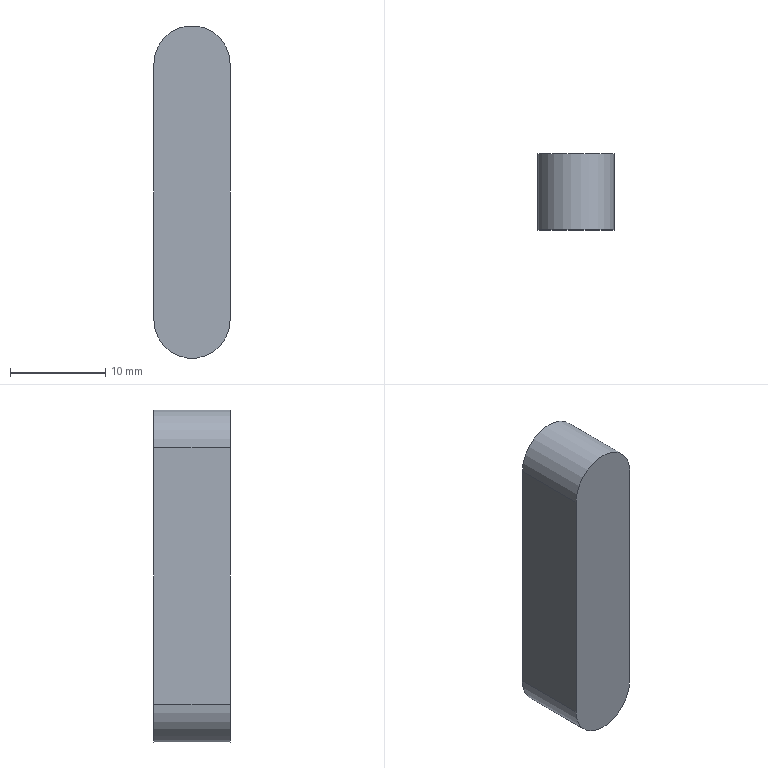Component | NX | FLAT_KEY_2 | 1 solid | 6 faces | box 8 x 8 x 35 mm | volume 2130 mm3 | plane 4 | cylinder 2 | commonest cylinder face diameters 8 x2
STEP:
#1=CARTESIAN_POINT('',(0.,0.,0.));
#2=DIRECTION('',(0.,0.,1.));
#3=DIRECTION('',(1.,0.,0.));
#4=AXIS2_PLACEMENT_3D('',#1,#2,#3);
#5=CARTESIAN_POINT('',(-515.175,316.681,-714.));
#6=VERTEX_POINT('',#5);
#7=CARTESIAN_POINT('',(-515.175,316.681,-687.));
#8=VERTEX_POINT('',#7);
#9=CARTESIAN_POINT('',(-515.175,316.681,-700.5));
#10=DIRECTION('',(0.,0.,1.));
#11=VECTOR('',#10,1.);
#12=LINE('',#9,#11);
#13=CARTESIAN_POINT('',(-511.175,316.681,-700.5));
#14=DIRECTION('',(0.,-1.,0.));
#15=DIRECTION('',(0.,0.,-1.));
#16=AXIS2_PLACEMENT_3D('',#13,#14,#15);
#17=PLANE('',#16);
#18=CARTESIAN_POINT('',(0.,-4.));
#19=DIRECTION('',(-1.,0.));
#20=VECTOR('',#19,1.);
#21=LINE('',#18,#20);
#22=(GEOMETRIC_REPRESENTATION_CONTEXT(2)PARAMETRIC_REPRESENTATION_CONTEXT()REPRESENTATION_CONTEXT('',''));
#23=DEFINITIONAL_REPRESENTATION('',(#21),#22);
#24=PCURVE('',#17,#23);
#25=CARTESIAN_POINT('',(-515.175,324.681,-700.5));
#26=DIRECTION('',(-1.,0.,0.));
#27=DIRECTION('',(0.,1.,0.));
#28=AXIS2_PLACEMENT_3D('',#25,#26,#27);
#29=PLANE('',#28);
#30=CARTESIAN_POINT('',(-8.,0.));
#31=DIRECTION('',(0.,-1.));
#32=VECTOR('',#31,1.);
#33=LINE('',#30,#32);
#34=(GEOMETRIC_REPRESENTATION_CONTEXT(2)PARAMETRIC_REPRESENTATION_CONTEXT()REPRESENTATION_CONTEXT('',''));
#35=DEFINITIONAL_REPRESENTATION('',(#33),#34);
#36=PCURVE('',#29,#35);
#37=SURFACE_CURVE('',#12,(#24,#36),.PCURVE_S1.);
#38=EDGE_CURVE('',#6,#8,#37,.T.);
#39=ORIENTED_EDGE('',*,*,#38,.F.);
#40=CARTESIAN_POINT('',(-507.175,316.681,-714.));
#41=VERTEX_POINT('',#40);
#42=CARTESIAN_POINT('',(-511.175,316.681,-714.));
#43=DIRECTION('',(0.,-1.,0.));
#44=DIRECTION('',(0.,0.,-1.));
#45=AXIS2_PLACEMENT_3D('',#42,#43,#44);
#46=CIRCLE('',#45,4.);
#47=CARTESIAN_POINT('',(13.5,0.));
#48=DIRECTION('',(1.,0.));
#49=AXIS2_PLACEMENT_2D('',#47,#48);
#50=CIRCLE('',#49,4.);
#51=(GEOMETRIC_REPRESENTATION_CONTEXT(2)PARAMETRIC_REPRESENTATION_CONTEXT()REPRESENTATION_CONTEXT('',''));
#52=DEFINITIONAL_REPRESENTATION('',(#50),#51);
#53=PCURVE('',#17,#52);
#54=CARTESIAN_POINT('',(-511.175,324.681,-714.));
#55=DIRECTION('',(0.,-1.,0.));
#56=DIRECTION('',(0.,0.,-1.));
#57=AXIS2_PLACEMENT_3D('',#54,#55,#56);
#58=CYLINDRICAL_SURFACE('',#57,4.);
#59=CARTESIAN_POINT('',(0.,8.));
#60=DIRECTION('',(1.,0.));
#61=VECTOR('',#60,1.);
#62=LINE('',#59,#61);
#63=(GEOMETRIC_REPRESENTATION_CONTEXT(2)PARAMETRIC_REPRESENTATION_CONTEXT()REPRESENTATION_CONTEXT('',''));
#64=DEFINITIONAL_REPRESENTATION('',(#62),#63);
#65=PCURVE('',#58,#64);
#66=SURFACE_CURVE('',#46,(#53,#65),.PCURVE_S1.);
#67=EDGE_CURVE('',#6,#41,#66,.T.);
#68=ORIENTED_EDGE('',*,*,#67,.T.);
#69=CARTESIAN_POINT('',(-507.175,316.681,-687.));
#70=VERTEX_POINT('',#69);
#71=CARTESIAN_POINT('',(-507.175,316.681,-700.5));
#72=DIRECTION('',(0.,0.,-1.));
#73=VECTOR('',#72,1.);
#74=LINE('',#71,#73);
#75=CARTESIAN_POINT('',(0.,4.));
#76=DIRECTION('',(1.,0.));
#77=VECTOR('',#76,1.);
#78=LINE('',#75,#77);
#79=(GEOMETRIC_REPRESENTATION_CONTEXT(2)PARAMETRIC_REPRESENTATION_CONTEXT()REPRESENTATION_CONTEXT('',''));
#80=DEFINITIONAL_REPRESENTATION('',(#78),#79);
#81=PCURVE('',#17,#80);
#82=CARTESIAN_POINT('',(-507.175,324.681,-700.5));
#83=DIRECTION('',(1.,0.,0.));
#84=DIRECTION('',(0.,-1.,0.));
#85=AXIS2_PLACEMENT_3D('',#82,#83,#84);
#86=PLANE('',#85);
#87=CARTESIAN_POINT('',(8.,0.));
#88=DIRECTION('',(0.,1.));
#89=VECTOR('',#88,1.);
#90=LINE('',#87,#89);
#91=(GEOMETRIC_REPRESENTATION_CONTEXT(2)PARAMETRIC_REPRESENTATION_CONTEXT()REPRESENTATION_CONTEXT('',''));
#92=DEFINITIONAL_REPRESENTATION('',(#90),#91);
#93=PCURVE('',#86,#92);
#94=SURFACE_CURVE('',#74,(#81,#93),.PCURVE_S1.);
#95=EDGE_CURVE('',#70,#41,#94,.T.);
#96=ORIENTED_EDGE('',*,*,#95,.F.);
#97=CARTESIAN_POINT('',(-511.175,316.681,-687.));
#98=DIRECTION('',(0.,-1.,0.));
#99=DIRECTION('',(0.,0.,-1.));
#100=AXIS2_PLACEMENT_3D('',#97,#98,#99);
#101=CIRCLE('',#100,4.);
#102=CARTESIAN_POINT('',(-13.5,0.));
#103=DIRECTION('',(1.,0.));
#104=AXIS2_PLACEMENT_2D('',#102,#103);
#105=CIRCLE('',#104,4.);
#106=(GEOMETRIC_REPRESENTATION_CONTEXT(2)PARAMETRIC_REPRESENTATION_CONTEXT()REPRESENTATION_CONTEXT('',''));
#107=DEFINITIONAL_REPRESENTATION('',(#105),#106);
#108=PCURVE('',#17,#107);
#109=CARTESIAN_POINT('',(-511.175,324.681,-687.));
#110=DIRECTION('',(0.,-1.,0.));
#111=DIRECTION('',(0.,0.,-1.));
#112=AXIS2_PLACEMENT_3D('',#109,#110,#111);
#113=CYLINDRICAL_SURFACE('',#112,4.);
#114=CARTESIAN_POINT('',(0.,8.));
#115=DIRECTION('',(1.,0.));
#116=VECTOR('',#115,1.);
#117=LINE('',#114,#116);
#118=(GEOMETRIC_REPRESENTATION_CONTEXT(2)PARAMETRIC_REPRESENTATION_CONTEXT()REPRESENTATION_CONTEXT('',''));
#119=DEFINITIONAL_REPRESENTATION('',(#117),#118);
#120=PCURVE('',#113,#119);
#121=SURFACE_CURVE('',#101,(#108,#120),.PCURVE_S1.);
#122=EDGE_CURVE('',#70,#8,#121,.T.);
#123=ORIENTED_EDGE('',*,*,#122,.T.);
#124=EDGE_LOOP('',(#39,#68,#96,#123));
#125=FACE_BOUND('',#124,.T.);
#126=ADVANCED_FACE('',(#125),#17,.T.);
#127=CARTESIAN_POINT('',(-515.175,324.681,-687.));
#128=VERTEX_POINT('',#127);
#129=CARTESIAN_POINT('',(-515.175,324.681,-714.));
#130=VERTEX_POINT('',#129);
#131=CARTESIAN_POINT('',(-515.175,324.681,-700.5));
#132=DIRECTION('',(0.,0.,-1.));
#133=VECTOR('',#132,1.);
#134=LINE('',#131,#133);
#135=CARTESIAN_POINT('',(0.,0.));
#136=DIRECTION('',(0.,1.));
#137=VECTOR('',#136,1.);
#138=LINE('',#135,#137);
#139=(GEOMETRIC_REPRESENTATION_CONTEXT(2)PARAMETRIC_REPRESENTATION_CONTEXT()REPRESENTATION_CONTEXT('',''));
#140=DEFINITIONAL_REPRESENTATION('',(#138),#139);
#141=PCURVE('',#29,#140);
#142=CARTESIAN_POINT('',(-511.175,324.681,-700.5));
#143=DIRECTION('',(0.,1.,0.));
#144=DIRECTION('',(0.,0.,1.));
#145=AXIS2_PLACEMENT_3D('',#142,#143,#144);
#146=PLANE('',#145);
#147=CARTESIAN_POINT('',(0.,-4.));
#148=DIRECTION('',(-1.,0.));
#149=VECTOR('',#148,1.);
#150=LINE('',#147,#149);
#151=(GEOMETRIC_REPRESENTATION_CONTEXT(2)PARAMETRIC_REPRESENTATION_CONTEXT()REPRESENTATION_CONTEXT('',''));
#152=DEFINITIONAL_REPRESENTATION('',(#150),#151);
#153=PCURVE('',#146,#152);
#154=SURFACE_CURVE('',#134,(#141,#153),.PCURVE_S1.);
#155=EDGE_CURVE('',#128,#130,#154,.T.);
#156=ORIENTED_EDGE('',*,*,#155,.T.);
#157=CARTESIAN_POINT('',(-515.175,324.681,-714.));
#158=DIRECTION('',(0.,-1.,0.));
#159=VECTOR('',#158,1.);
#160=LINE('',#157,#159);
#161=CARTESIAN_POINT('',(0.,13.5));
#162=DIRECTION('',(-1.,0.));
#163=VECTOR('',#162,1.);
#164=LINE('',#161,#163);
#165=(GEOMETRIC_REPRESENTATION_CONTEXT(2)PARAMETRIC_REPRESENTATION_CONTEXT()REPRESENTATION_CONTEXT('',''));
#166=DEFINITIONAL_REPRESENTATION('',(#164),#165);
#167=PCURVE('',#29,#166);
#168=CARTESIAN_POINT('',(4.712,0.));
#169=DIRECTION('',(0.,1.));
#170=VECTOR('',#169,1.);
#171=LINE('',#168,#170);
#172=(GEOMETRIC_REPRESENTATION_CONTEXT(2)PARAMETRIC_REPRESENTATION_CONTEXT()REPRESENTATION_CONTEXT('',''));
#173=DEFINITIONAL_REPRESENTATION('',(#171),#172);
#174=PCURVE('',#58,#173);
#175=SURFACE_CURVE('',#160,(#167,#174),.PCURVE_S1.);
#176=EDGE_CURVE('',#130,#6,#175,.T.);
#177=ORIENTED_EDGE('',*,*,#176,.T.);
#178=ORIENTED_EDGE('',*,*,#38,.T.);
#179=CARTESIAN_POINT('',(-515.175,324.681,-687.));
#180=DIRECTION('',(0.,1.,0.));
#181=VECTOR('',#180,1.);
#182=LINE('',#179,#181);
#183=CARTESIAN_POINT('',(0.,-13.5));
#184=DIRECTION('',(1.,0.));
#185=VECTOR('',#184,1.);
#186=LINE('',#183,#185);
#187=(GEOMETRIC_REPRESENTATION_CONTEXT(2)PARAMETRIC_REPRESENTATION_CONTEXT()REPRESENTATION_CONTEXT('',''));
#188=DEFINITIONAL_REPRESENTATION('',(#186),#187);
#189=PCURVE('',#29,#188);
#190=CARTESIAN_POINT('',(4.712,0.));
#191=DIRECTION('',(0.,-1.));
#192=VECTOR('',#191,1.);
#193=LINE('',#190,#192);
#194=(GEOMETRIC_REPRESENTATION_CONTEXT(2)PARAMETRIC_REPRESENTATION_CONTEXT()REPRESENTATION_CONTEXT('',''));
#195=DEFINITIONAL_REPRESENTATION('',(#193),#194);
#196=PCURVE('',#113,#195);
#197=SURFACE_CURVE('',#182,(#189,#196),.PCURVE_S1.);
#198=EDGE_CURVE('',#8,#128,#197,.T.);
#199=ORIENTED_EDGE('',*,*,#198,.T.);
#200=EDGE_LOOP('',(#156,#177,#178,#199));
#201=FACE_BOUND('',#200,.T.);
#202=ADVANCED_FACE('',(#201),#29,.T.);
#203=ORIENTED_EDGE('',*,*,#95,.T.);
#204=CARTESIAN_POINT('',(-507.175,324.681,-714.));
#205=VERTEX_POINT('',#204);
#206=CARTESIAN_POINT('',(-507.175,324.681,-714.));
#207=DIRECTION('',(0.,1.,0.));
#208=VECTOR('',#207,1.);
#209=LINE('',#206,#208);
#210=CARTESIAN_POINT('',(0.,13.5));
#211=DIRECTION('',(-1.,0.));
#212=VECTOR('',#211,1.);
#213=LINE('',#210,#212);
#214=(GEOMETRIC_REPRESENTATION_CONTEXT(2)PARAMETRIC_REPRESENTATION_CONTEXT()REPRESENTATION_CONTEXT('',''));
#215=DEFINITIONAL_REPRESENTATION('',(#213),#214);
#216=PCURVE('',#86,#215);
#217=CARTESIAN_POINT('',(7.854,0.));
#218=DIRECTION('',(0.,-1.));
#219=VECTOR('',#218,1.);
#220=LINE('',#217,#219);
#221=(GEOMETRIC_REPRESENTATION_CONTEXT(2)PARAMETRIC_REPRESENTATION_CONTEXT()REPRESENTATION_CONTEXT('',''));
#222=DEFINITIONAL_REPRESENTATION('',(#220),#221);
#223=PCURVE('',#58,#222);
#224=SURFACE_CURVE('',#209,(#216,#223),.PCURVE_S1.);
#225=EDGE_CURVE('',#41,#205,#224,.T.);
#226=ORIENTED_EDGE('',*,*,#225,.T.);
#227=CARTESIAN_POINT('',(-507.175,324.681,-687.));
#228=VERTEX_POINT('',#227);
#229=CARTESIAN_POINT('',(-507.175,324.681,-700.5));
#230=DIRECTION('',(0.,0.,1.));
#231=VECTOR('',#230,1.);
#232=LINE('',#229,#231);
#233=CARTESIAN_POINT('',(0.,0.));
#234=DIRECTION('',(0.,-1.));
#235=VECTOR('',#234,1.);
#236=LINE('',#233,#235);
#237=(GEOMETRIC_REPRESENTATION_CONTEXT(2)PARAMETRIC_REPRESENTATION_CONTEXT()REPRESENTATION_CONTEXT('',''));
#238=DEFINITIONAL_REPRESENTATION('',(#236),#237);
#239=PCURVE('',#86,#238);
#240=CARTESIAN_POINT('',(0.,4.));
#241=DIRECTION('',(1.,0.));
#242=VECTOR('',#241,1.);
#243=LINE('',#240,#242);
#244=(GEOMETRIC_REPRESENTATION_CONTEXT(2)PARAMETRIC_REPRESENTATION_CONTEXT()REPRESENTATION_CONTEXT('',''));
#245=DEFINITIONAL_REPRESENTATION('',(#243),#244);
#246=PCURVE('',#146,#245);
#247=SURFACE_CURVE('',#232,(#239,#246),.PCURVE_S1.);
#248=EDGE_CURVE('',#205,#228,#247,.T.);
#249=ORIENTED_EDGE('',*,*,#248,.T.);
#250=CARTESIAN_POINT('',(-507.175,324.681,-687.));
#251=DIRECTION('',(0.,-1.,0.));
#252=VECTOR('',#251,1.);
#253=LINE('',#250,#252);
#254=CARTESIAN_POINT('',(0.,-13.5));
#255=DIRECTION('',(1.,0.));
#256=VECTOR('',#255,1.);
#257=LINE('',#254,#256);
#258=(GEOMETRIC_REPRESENTATION_CONTEXT(2)PARAMETRIC_REPRESENTATION_CONTEXT()REPRESENTATION_CONTEXT('',''));
#259=DEFINITIONAL_REPRESENTATION('',(#257),#258);
#260=PCURVE('',#86,#259);
#261=CARTESIAN_POINT('',(1.571,0.));
#262=DIRECTION('',(0.,1.));
#263=VECTOR('',#262,1.);
#264=LINE('',#261,#263);
#265=(GEOMETRIC_REPRESENTATION_CONTEXT(2)PARAMETRIC_REPRESENTATION_CONTEXT()REPRESENTATION_CONTEXT('',''));
#266=DEFINITIONAL_REPRESENTATION('',(#264),#265);
#267=PCURVE('',#113,#266);
#268=SURFACE_CURVE('',#253,(#260,#267),.PCURVE_S1.);
#269=EDGE_CURVE('',#228,#70,#268,.T.);
#270=ORIENTED_EDGE('',*,*,#269,.T.);
#271=EDGE_LOOP('',(#203,#226,#249,#270));
#272=FACE_BOUND('',#271,.T.);
#273=ADVANCED_FACE('',(#272),#86,.T.);
#274=CARTESIAN_POINT('',(-511.175,324.681,-714.));
#275=DIRECTION('',(0.,1.,0.));
#276=DIRECTION('',(0.,0.,1.));
#277=AXIS2_PLACEMENT_3D('',#274,#275,#276);
#278=CIRCLE('',#277,4.);
#279=CARTESIAN_POINT('',(-13.5,0.));
#280=DIRECTION('',(1.,0.));
#281=AXIS2_PLACEMENT_2D('',#279,#280);
#282=CIRCLE('',#281,4.);
#283=(GEOMETRIC_REPRESENTATION_CONTEXT(2)PARAMETRIC_REPRESENTATION_CONTEXT()REPRESENTATION_CONTEXT('',''));
#284=DEFINITIONAL_REPRESENTATION('',(#282),#283);
#285=PCURVE('',#146,#284);
#286=CARTESIAN_POINT('',(9.425,0.));
#287=DIRECTION('',(-1.,0.));
#288=VECTOR('',#287,1.);
#289=LINE('',#286,#288);
#290=(GEOMETRIC_REPRESENTATION_CONTEXT(2)PARAMETRIC_REPRESENTATION_CONTEXT()REPRESENTATION_CONTEXT('',''));
#291=DEFINITIONAL_REPRESENTATION('',(#289),#290);
#292=PCURVE('',#58,#291);
#293=SURFACE_CURVE('',#278,(#285,#292),.PCURVE_S1.);
#294=EDGE_CURVE('',#205,#130,#293,.T.);
#295=ORIENTED_EDGE('',*,*,#294,.T.);
#296=ORIENTED_EDGE('',*,*,#155,.F.);
#297=CARTESIAN_POINT('',(-511.175,324.681,-687.));
#298=DIRECTION('',(0.,1.,0.));
#299=DIRECTION('',(0.,0.,1.));
#300=AXIS2_PLACEMENT_3D('',#297,#298,#299);
#301=CIRCLE('',#300,4.);
#302=CARTESIAN_POINT('',(13.5,0.));
#303=DIRECTION('',(1.,0.));
#304=AXIS2_PLACEMENT_2D('',#302,#303);
#305=CIRCLE('',#304,4.);
#306=(GEOMETRIC_REPRESENTATION_CONTEXT(2)PARAMETRIC_REPRESENTATION_CONTEXT()REPRESENTATION_CONTEXT('',''));
#307=DEFINITIONAL_REPRESENTATION('',(#305),#306);
#308=PCURVE('',#146,#307);
#309=CARTESIAN_POINT('',(9.425,0.));
#310=DIRECTION('',(-1.,0.));
#311=VECTOR('',#310,1.);
#312=LINE('',#309,#311);
#313=(GEOMETRIC_REPRESENTATION_CONTEXT(2)PARAMETRIC_REPRESENTATION_CONTEXT()REPRESENTATION_CONTEXT('',''));
#314=DEFINITIONAL_REPRESENTATION('',(#312),#313);
#315=PCURVE('',#113,#314);
#316=SURFACE_CURVE('',#301,(#308,#315),.PCURVE_S1.);
#317=EDGE_CURVE('',#128,#228,#316,.T.);
#318=ORIENTED_EDGE('',*,*,#317,.T.);
#319=ORIENTED_EDGE('',*,*,#248,.F.);
#320=EDGE_LOOP('',(#295,#296,#318,#319));
#321=FACE_BOUND('',#320,.T.);
#322=ADVANCED_FACE('',(#321),#146,.T.);
#323=ORIENTED_EDGE('',*,*,#67,.F.);
#324=ORIENTED_EDGE('',*,*,#176,.F.);
#325=ORIENTED_EDGE('',*,*,#294,.F.);
#326=ORIENTED_EDGE('',*,*,#225,.F.);
#327=EDGE_LOOP('',(#323,#324,#325,#326));
#328=FACE_BOUND('',#327,.T.);
#329=ADVANCED_FACE('',(#328),#58,.T.);
#330=ORIENTED_EDGE('',*,*,#122,.F.);
#331=ORIENTED_EDGE('',*,*,#269,.F.);
#332=ORIENTED_EDGE('',*,*,#317,.F.);
#333=ORIENTED_EDGE('',*,*,#198,.F.);
#334=EDGE_LOOP('',(#330,#331,#332,#333));
#335=FACE_BOUND('',#334,.T.);
#336=ADVANCED_FACE('',(#335),#113,.T.);
#337=CLOSED_SHELL('',(#126,#202,#273,#322,#329,#336));
#338=MANIFOLD_SOLID_BREP('',#337);
#339=(LENGTH_UNIT()NAMED_UNIT(*)SI_UNIT(.MILLI.,.METRE.));
#340=UNCERTAINTY_MEASURE_WITH_UNIT(LENGTH_MEASURE(0.0000001),#339,'','');
#341=(NAMED_UNIT(*)PLANE_ANGLE_UNIT()SI_UNIT($,.RADIAN.));
#342=(NAMED_UNIT(*)SI_UNIT($,.STERADIAN.)SOLID_ANGLE_UNIT());
#343=(GEOMETRIC_REPRESENTATION_CONTEXT(3)GLOBAL_UNCERTAINTY_ASSIGNED_CONTEXT((#340))GLOBAL_UNIT_ASSIGNED_CONTEXT((#339,#341,#342))REPRESENTATION_CONTEXT('',''));
#344=ADVANCED_BREP_SHAPE_REPRESENTATION('',(#4,#338),#343);